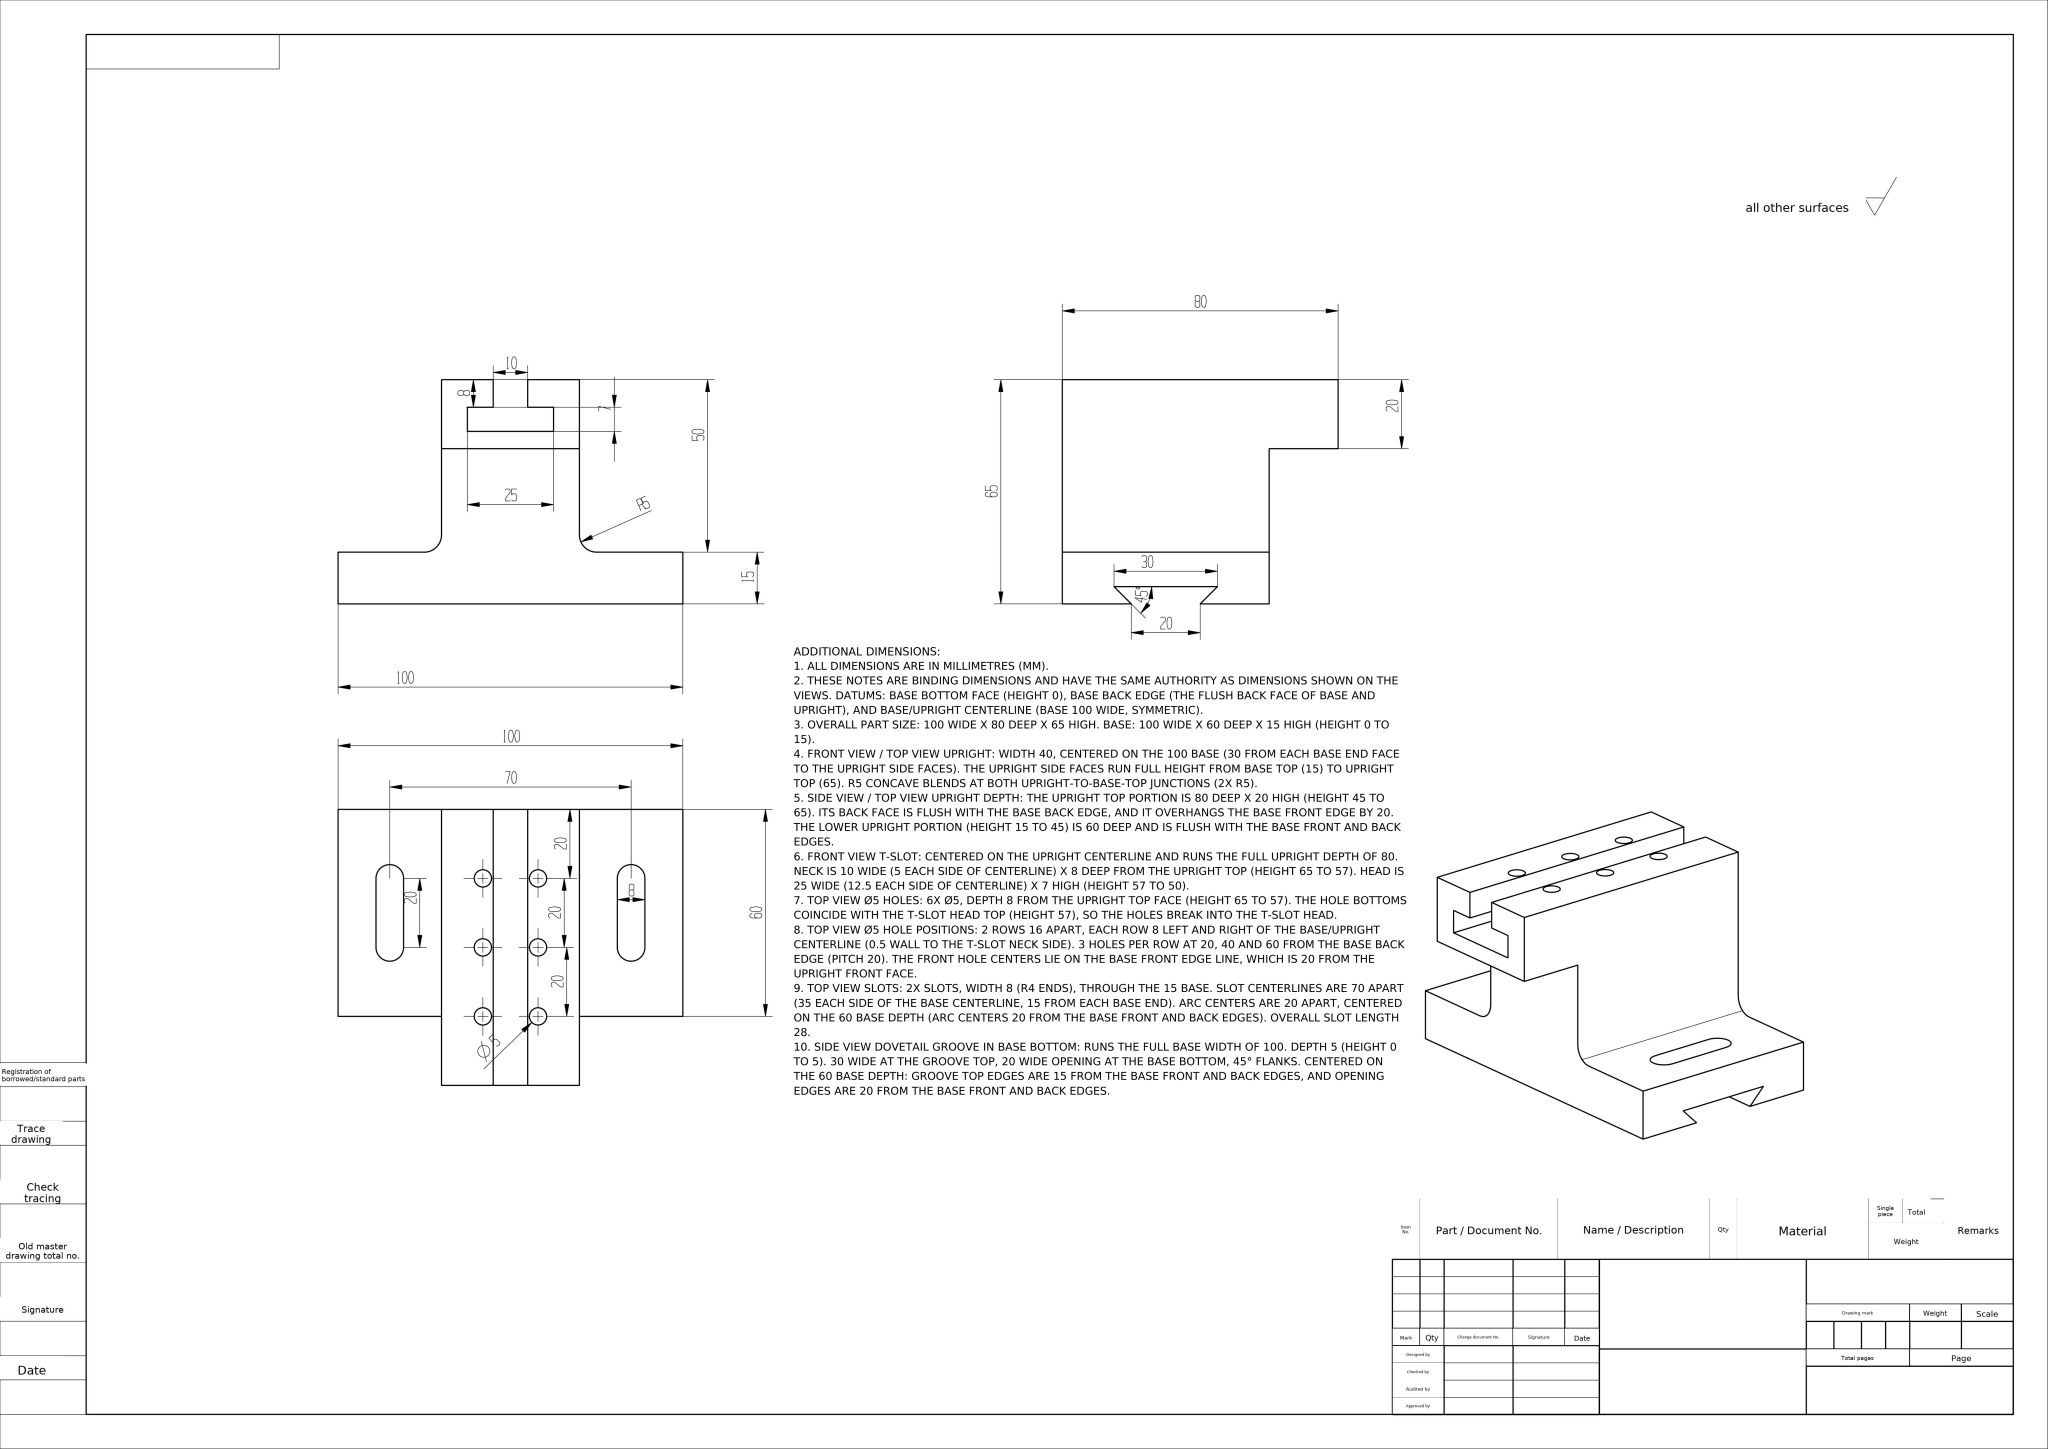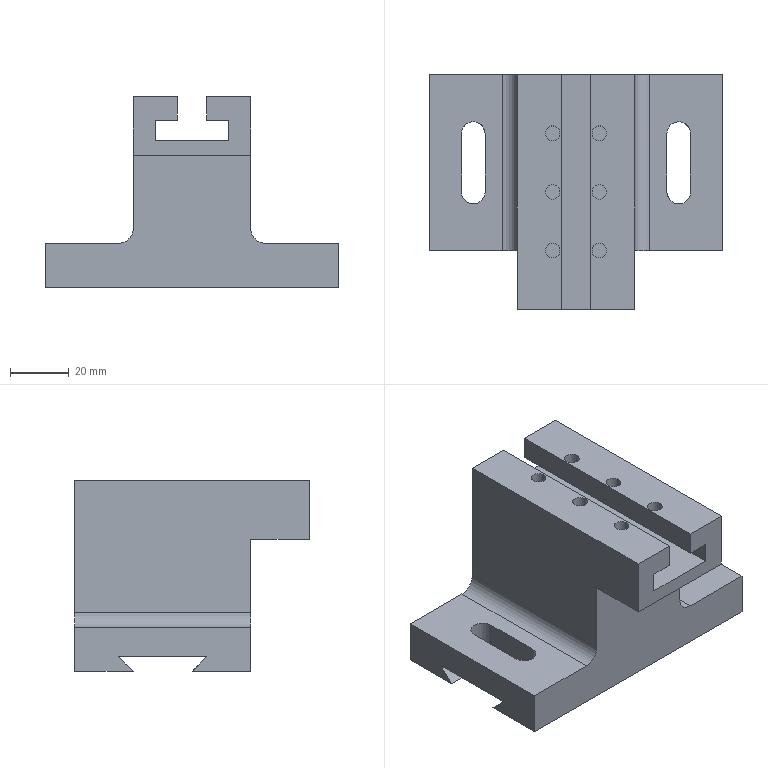Part | NX | mm | 1 solid | 44 faces | box 100 x 80 x 65 mm | volume 188425 mm3 | plane 28 | cylinder 16 | commonest cylinder face diameters 8 x8 5 x6 10 x2